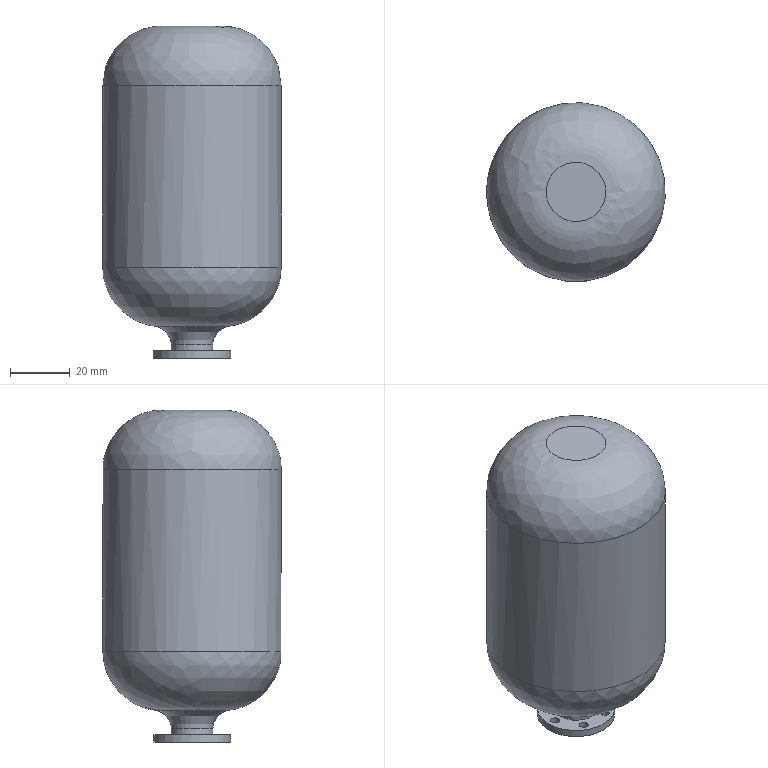Component | NX | WATER_CHAMBER | 1 solid | 21 faces | volume 41306 mm3 | cylinder 11 | plane 4 | spline 4 | torus 2 | commonest cylinder face diameters 3 x6 26 x1 60 x1 14 x1 56 x1 10 x1